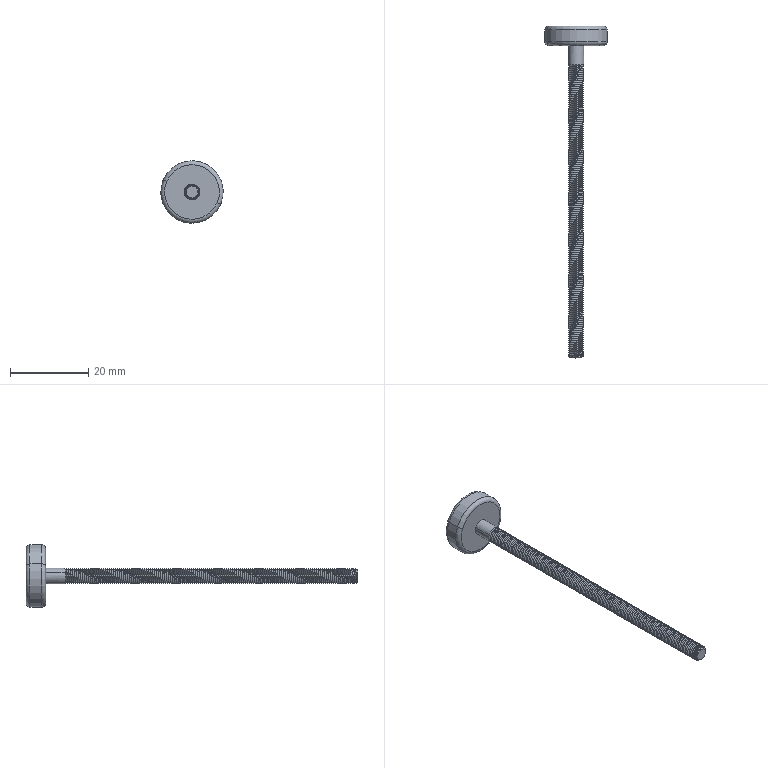Component | SolidWorks | LongBoltM4.1-1 | 1 solid | 315 faces | volume 1795 mm3 | cylinder 302 | torus 4 | plane 4 | cone 3 | spline 2 | commonest cylinder face diameters 4 x300 16 x2